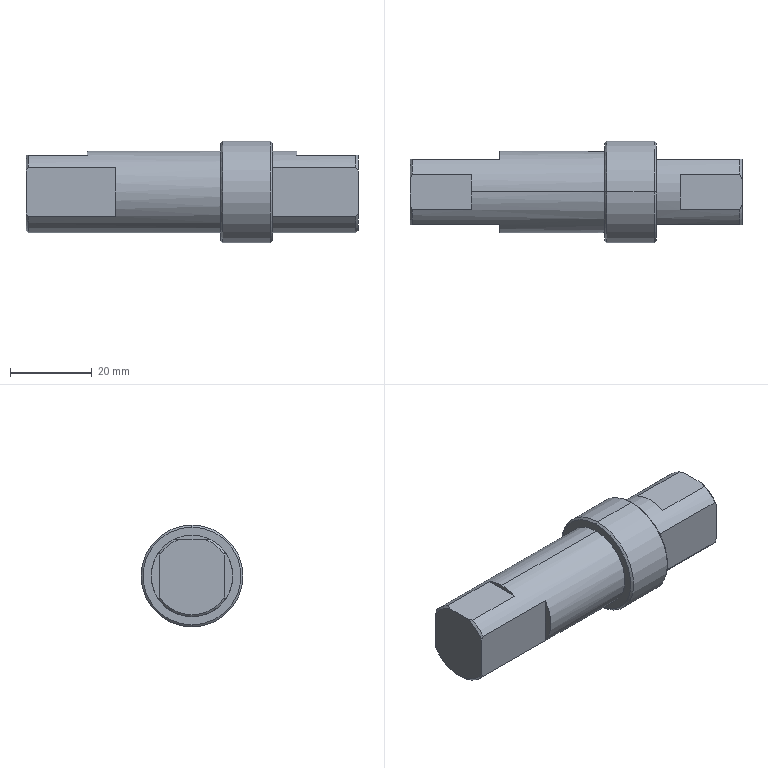Component | SolidWorks | ChainPartDrivenShaft-1 | 1 solid | 32 faces | box 81.4 x 25 x 25 mm | volume 26208 mm3 | plane 14 | cone 11 | cylinder 7 | commonest cylinder face diameters 20 x5 25 x2
build123d program:
from build123d import *

# Parameters (mm, degrees)
CHAMFER1_SIZE           = 0.5
SKETCH2_W               = 2
SKETCH2_H               = 21
SKETCH2_H_2             = 22
CUT_EXTRUDE1_DEPTH      = 20
CUT_EXTRUDE2_DEPTH      = 84.297
CUT_EXTRUDE2_DEPTH_BACK = 84.297
SKETCH3_W               = 1
SKETCH3_H               = 15


with BuildPart() as part:
    # Sketch1 → Revolve1 (revolve)
    with BuildSketch(Plane.XY, mode=Mode.PRIVATE) as revolve1_sk:
        Polygon((0, 0), (10, 0), (10, 47.7), (12.5, 47.7), (12.5, 60.4), (10, 60.4), (10, 81.4), (0, 81.4), align=None)
    revolve(revolve1_sk.sketch.rotate(Axis((0, 0, 0), (0, 1, 0)), 90), axis=Axis((0, 0, 0), (0, 1, 0)))

    # Chamfer1
    chamfer1_edges = [part.edges().sort_by_distance(p)[0] for p in [
        (0, 81.4, 10),
        (0, 60.4, 12.5),
        (0, 47.7, 12.5),
        (0, 0, 10),
    ]]
    chamfer(chamfer1_edges, length=CHAMFER1_SIZE)

    # Sketch2 → Cut-Extrude1 (cut, symmetric)
    with BuildSketch(Plane.XY):
        with Locations((-9, 70.9)):
            Rectangle(SKETCH2_W, SKETCH2_H)
        with Locations((9, 70.9)):
            Rectangle(SKETCH2_W, SKETCH2_H)
        with Locations((-9, 11)):
            Rectangle(SKETCH2_W, SKETCH2_H_2)
        with Locations((9, 11)):
            Rectangle(SKETCH2_W, SKETCH2_H_2)
    extrude(amount=CUT_EXTRUDE1_DEPTH, both=True, mode=Mode.SUBTRACT)

    # Sketch3 → Cut-Extrude2 (cut, two sides: drawn at the far end of the back side and taken through both)
    with BuildSketch(Plane(origin=(0, 0, 0), x_dir=(0, 0, -1), z_dir=(1, 0, 0)).offset(-CUT_EXTRUDE2_DEPTH_BACK)):
        with Locations((-9.5, 73.9)):
            Rectangle(SKETCH3_W, SKETCH3_H)
        with Locations((-9.5, 7.5)):
            Rectangle(SKETCH3_W, SKETCH3_H)
    extrude(amount=CUT_EXTRUDE2_DEPTH + CUT_EXTRUDE2_DEPTH_BACK, mode=Mode.SUBTRACT)


solid = part.part

# Placed as in the assembly
solid = solid.moved(Location((67.237, -2.563, -673.885), (0, 0, -90)))